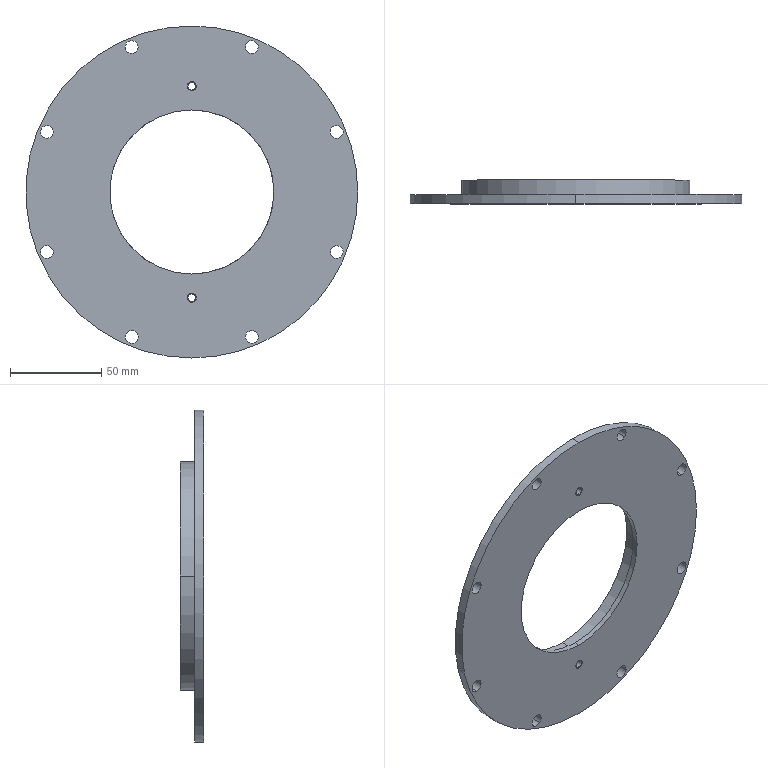CAM job | Mastercam | mm | 1 operations | part box 182 x 13 x 182
1. Drill/Counterbore | 5 - 4 倒角刀